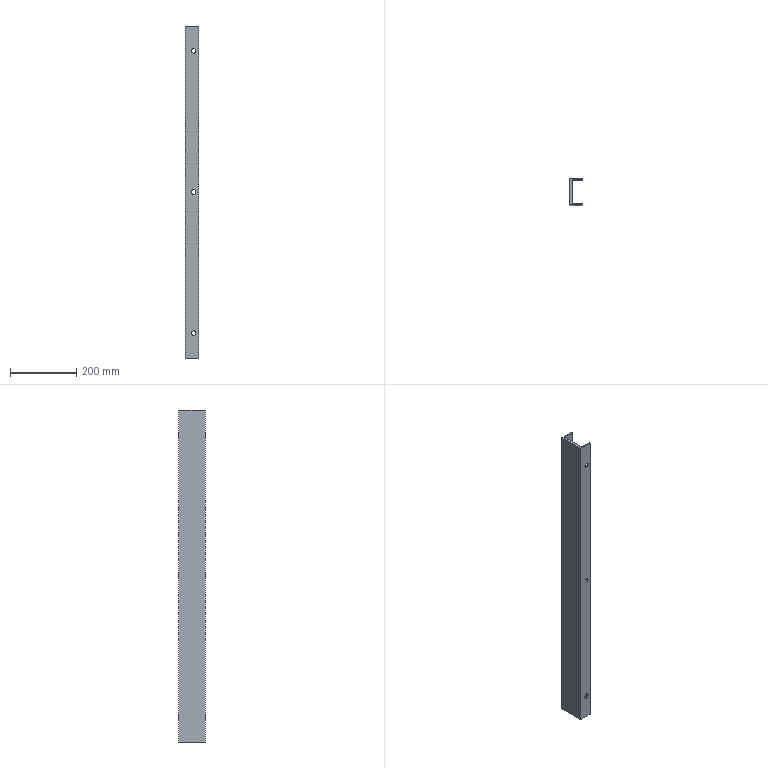Component | SolidWorks | BaseAssembly-1_ChannelSteelAssembly-1_8#ChannelSteel1-1 | 1 solid | 22 faces | box 40 x 80 x 1000 mm | volume 892305 mm3 | cylinder 12 | plane 10 | commonest cylinder face diameters 14 x12
build123d program:
from build123d import *

# Parameters (mm, degrees)
EXTRUDE1_DEPTH     = 1000
SKETCH2_R          = 7
CUT_EXTRUDE1_DEPTH = 1004.992
LPATTERN1_COUNT    = 3
LPATTERN1_PITCH    = 425


with BuildPart() as part:
    # Sketch1 → Extrude1 (new body)
    with BuildSketch(Plane.XY):
        Polygon((0, 0), (-40, 0), (-40, 80), (0, 80), (0, 76), (-32, 76), (-32, 4), (0, 4), align=None)
    extrude(amount=EXTRUDE1_DEPTH)

    # Sketch2 → Cut-Extrude1 (cut, through all)
    with BuildSketch(Plane(origin=(0, 80, 0), x_dir=(1, 0, 0), z_dir=(0, 1, 0))):
        with Locations(Location((-15, -925, 0), (0, 0, 270))):
            Circle(SKETCH2_R)
    cut_extrude1 = extrude(amount=-CUT_EXTRUDE1_DEPTH, mode=Mode.SUBTRACT)

    # LPattern1: Cut-Extrude1 ×3
    with Locations(*[(0, 0, -i * LPATTERN1_PITCH) for i in range(1, LPATTERN1_COUNT)]):
        add(cut_extrude1, mode=Mode.SUBTRACT)


solid = part.part

# Placed as in the assembly
solid = solid.moved(Location((-377.218, -82.9, -600), (0, 0, 0)))
STEP:
#1=COLOUR_RGB('',0.7922,0.8196,0.9333);
#2=FILL_AREA_STYLE_COLOUR('',#1);
#3=FILL_AREA_STYLE('',(#2));
#4=SURFACE_STYLE_FILL_AREA(#3);
#5=SURFACE_SIDE_STYLE('',(#4));
#6=SURFACE_STYLE_USAGE(.BOTH.,#5);
#7=PRESENTATION_STYLE_ASSIGNMENT((#6));
#8=CARTESIAN_POINT('',(-15.442,-3.264,-20.945));
#9=VERTEX_POINT('',#8);
#10=CARTESIAN_POINT('',(-15.442,-3.264,-20.394));
#11=VERTEX_POINT('',#10);
#12=CARTESIAN_POINT('',(-15.442,-3.264,-20.669));
#13=DIRECTION('',(0.,1.,0.));
#14=DIRECTION('',(0.,0.,1.));
#15=AXIS2_PLACEMENT_3D('',#12,#13,#14);
#16=CIRCLE('',#15,0.2756);
#17=EDGE_CURVE('',#9,#11,#16,.T.);
#18=ORIENTED_EDGE('',*,*,#17,.F.);
#19=CARTESIAN_POINT('',(-15.442,-3.106,-20.945));
#20=VERTEX_POINT('',#19);
#21=CARTESIAN_POINT('',(-15.442,-3.264,-20.945));
#22=DIRECTION('',(0.,1.,0.));
#23=VECTOR('',#22,39.37);
#24=LINE('',#21,#23);
#25=EDGE_CURVE('',#9,#20,#24,.T.);
#26=ORIENTED_EDGE('',*,*,#25,.T.);
#27=CARTESIAN_POINT('',(-15.442,-3.106,-20.394));
#28=VERTEX_POINT('',#27);
#29=CARTESIAN_POINT('',(-15.442,-3.106,-20.669));
#30=DIRECTION('',(0.,-1.,0.));
#31=DIRECTION('',(0.,0.,-1.));
#32=AXIS2_PLACEMENT_3D('',#29,#30,#31);
#33=CIRCLE('',#32,0.2756);
#34=EDGE_CURVE('',#28,#20,#33,.T.);
#35=ORIENTED_EDGE('',*,*,#34,.F.);
#36=CARTESIAN_POINT('',(-15.442,-3.264,-20.394));
#37=DIRECTION('',(0.,1.,0.));
#38=VECTOR('',#37,39.37);
#39=LINE('',#36,#38);
#40=EDGE_CURVE('',#11,#28,#39,.T.);
#41=ORIENTED_EDGE('',*,*,#40,.F.);
#42=EDGE_LOOP('',(#18,#26,#35,#41));
#43=FACE_OUTER_BOUND('',#42,.T.);
#44=CARTESIAN_POINT('',(-15.442,-3.264,-20.669));
#45=DIRECTION('',(0.,1.,0.));
#46=DIRECTION('',(0.,0.,1.));
#47=AXIS2_PLACEMENT_3D('',#44,#45,#46);
#48=CYLINDRICAL_SURFACE('',#47,0.2756);
#49=ADVANCED_FACE('',(#43),#48,.F.);
#50=CARTESIAN_POINT('',(-15.442,-3.264,-4.213));
#51=VERTEX_POINT('',#50);
#52=CARTESIAN_POINT('',(-15.442,-3.264,-3.661));
#53=VERTEX_POINT('',#52);
#54=CARTESIAN_POINT('',(-15.442,-3.264,-3.937));
#55=DIRECTION('',(0.,1.,0.));
#56=DIRECTION('',(0.,0.,1.));
#57=AXIS2_PLACEMENT_3D('',#54,#55,#56);
#58=CIRCLE('',#57,0.2756);
#59=EDGE_CURVE('',#51,#53,#58,.T.);
#60=ORIENTED_EDGE('',*,*,#59,.F.);
#61=CARTESIAN_POINT('',(-15.442,-3.106,-4.213));
#62=VERTEX_POINT('',#61);
#63=CARTESIAN_POINT('',(-15.442,-3.264,-4.213));
#64=DIRECTION('',(0.,1.,0.));
#65=VECTOR('',#64,39.37);
#66=LINE('',#63,#65);
#67=EDGE_CURVE('',#51,#62,#66,.T.);
#68=ORIENTED_EDGE('',*,*,#67,.T.);
#69=CARTESIAN_POINT('',(-15.442,-3.106,-3.661));
#70=VERTEX_POINT('',#69);
#71=CARTESIAN_POINT('',(-15.442,-3.106,-3.937));
#72=DIRECTION('',(0.,-1.,0.));
#73=DIRECTION('',(0.,0.,-1.));
#74=AXIS2_PLACEMENT_3D('',#71,#72,#73);
#75=CIRCLE('',#74,0.2756);
#76=EDGE_CURVE('',#70,#62,#75,.T.);
#77=ORIENTED_EDGE('',*,*,#76,.F.);
#78=CARTESIAN_POINT('',(-15.442,-3.264,-3.661));
#79=DIRECTION('',(0.,1.,0.));
#80=VECTOR('',#79,39.37);
#81=LINE('',#78,#80);
#82=EDGE_CURVE('',#53,#70,#81,.T.);
#83=ORIENTED_EDGE('',*,*,#82,.F.);
#84=EDGE_LOOP('',(#60,#68,#77,#83));
#85=FACE_OUTER_BOUND('',#84,.T.);
#86=CARTESIAN_POINT('',(-15.442,-3.264,-3.937));
#87=DIRECTION('',(0.,1.,0.));
#88=DIRECTION('',(0.,0.,1.));
#89=AXIS2_PLACEMENT_3D('',#86,#87,#88);
#90=CYLINDRICAL_SURFACE('',#89,0.2756);
#91=ADVANCED_FACE('',(#85),#90,.F.);
#92=CARTESIAN_POINT('',(-15.442,-0.2717,-20.945));
#93=VERTEX_POINT('',#92);
#94=CARTESIAN_POINT('',(-15.442,-0.2717,-20.394));
#95=VERTEX_POINT('',#94);
#96=CARTESIAN_POINT('',(-15.442,-0.2717,-20.669));
#97=DIRECTION('',(0.,1.,0.));
#98=DIRECTION('',(0.,0.,1.));
#99=AXIS2_PLACEMENT_3D('',#96,#97,#98);
#100=CIRCLE('',#99,0.2756);
#101=EDGE_CURVE('',#93,#95,#100,.T.);
#102=ORIENTED_EDGE('',*,*,#101,.F.);
#103=CARTESIAN_POINT('',(-15.442,-0.1142,-20.945));
#104=VERTEX_POINT('',#103);
#105=CARTESIAN_POINT('',(-15.442,-3.264,-20.945));
#106=DIRECTION('',(0.,1.,0.));
#107=VECTOR('',#106,39.37);
#108=LINE('',#105,#107);
#109=EDGE_CURVE('',#93,#104,#108,.T.);
#110=ORIENTED_EDGE('',*,*,#109,.T.);
#111=CARTESIAN_POINT('',(-15.442,-0.1142,-20.394));
#112=VERTEX_POINT('',#111);
#113=CARTESIAN_POINT('',(-15.442,-0.1142,-20.669));
#114=DIRECTION('',(0.,1.,0.));
#115=DIRECTION('',(0.,0.,1.));
#116=AXIS2_PLACEMENT_3D('',#113,#114,#115);
#117=CIRCLE('',#116,0.2756);
#118=EDGE_CURVE('',#104,#112,#117,.T.);
#119=ORIENTED_EDGE('',*,*,#118,.T.);
#120=CARTESIAN_POINT('',(-15.442,-3.264,-20.394));
#121=DIRECTION('',(0.,1.,0.));
#122=VECTOR('',#121,39.37);
#123=LINE('',#120,#122);
#124=EDGE_CURVE('',#95,#112,#123,.T.);
#125=ORIENTED_EDGE('',*,*,#124,.F.);
#126=EDGE_LOOP('',(#102,#110,#119,#125));
#127=FACE_OUTER_BOUND('',#126,.T.);
#128=CARTESIAN_POINT('',(-15.442,-3.264,-20.669));
#129=DIRECTION('',(0.,1.,0.));
#130=DIRECTION('',(0.,0.,1.));
#131=AXIS2_PLACEMENT_3D('',#128,#129,#130);
#132=CYLINDRICAL_SURFACE('',#131,0.2756);
#133=ADVANCED_FACE('',(#127),#132,.F.);
#134=CARTESIAN_POINT('',(-15.442,-0.2717,-4.213));
#135=VERTEX_POINT('',#134);
#136=CARTESIAN_POINT('',(-15.442,-0.2717,-3.661));
#137=VERTEX_POINT('',#136);
#138=CARTESIAN_POINT('',(-15.442,-0.2717,-3.937));
#139=DIRECTION('',(0.,1.,0.));
#140=DIRECTION('',(0.,0.,1.));
#141=AXIS2_PLACEMENT_3D('',#138,#139,#140);
#142=CIRCLE('',#141,0.2756);
#143=EDGE_CURVE('',#135,#137,#142,.T.);
#144=ORIENTED_EDGE('',*,*,#143,.F.);
#145=CARTESIAN_POINT('',(-15.442,-0.1142,-4.213));
#146=VERTEX_POINT('',#145);
#147=CARTESIAN_POINT('',(-15.442,-3.264,-4.213));
#148=DIRECTION('',(0.,1.,0.));
#149=VECTOR('',#148,39.37);
#150=LINE('',#147,#149);
#151=EDGE_CURVE('',#135,#146,#150,.T.);
#152=ORIENTED_EDGE('',*,*,#151,.T.);
#153=CARTESIAN_POINT('',(-15.442,-0.1142,-3.661));
#154=VERTEX_POINT('',#153);
#155=CARTESIAN_POINT('',(-15.442,-0.1142,-3.937));
#156=DIRECTION('',(0.,1.,0.));
#157=DIRECTION('',(0.,0.,1.));
#158=AXIS2_PLACEMENT_3D('',#155,#156,#157);
#159=CIRCLE('',#158,0.2756);
#160=EDGE_CURVE('',#146,#154,#159,.T.);
#161=ORIENTED_EDGE('',*,*,#160,.T.);
#162=CARTESIAN_POINT('',(-15.442,-3.264,-3.661));
#163=DIRECTION('',(0.,1.,0.));
#164=VECTOR('',#163,39.37);
#165=LINE('',#162,#164);
#166=EDGE_CURVE('',#137,#154,#165,.T.);
#167=ORIENTED_EDGE('',*,*,#166,.F.);
#168=EDGE_LOOP('',(#144,#152,#161,#167));
#169=FACE_OUTER_BOUND('',#168,.T.);
#170=CARTESIAN_POINT('',(-15.442,-3.264,-3.937));
#171=DIRECTION('',(0.,1.,0.));
#172=DIRECTION('',(0.,0.,1.));
#173=AXIS2_PLACEMENT_3D('',#170,#171,#172);
#174=CYLINDRICAL_SURFACE('',#173,0.2756);
#175=ADVANCED_FACE('',(#169),#174,.F.);
#176=CARTESIAN_POINT('',(-15.442,-0.2717,12.52));
#177=VERTEX_POINT('',#176);
#178=CARTESIAN_POINT('',(-15.442,-0.2717,13.071));
#179=VERTEX_POINT('',#178);
#180=CARTESIAN_POINT('',(-15.442,-0.2717,12.795));
#181=DIRECTION('',(0.,1.,0.));
#182=DIRECTION('',(0.,0.,1.));
#183=AXIS2_PLACEMENT_3D('',#180,#181,#182);
#184=CIRCLE('',#183,0.2756);
#185=EDGE_CURVE('',#177,#179,#184,.T.);
#186=ORIENTED_EDGE('',*,*,#185,.F.);
#187=CARTESIAN_POINT('',(-15.442,-0.1142,12.52));
#188=VERTEX_POINT('',#187);
#189=CARTESIAN_POINT('',(-15.442,-3.264,12.52));
#190=DIRECTION('',(0.,1.,0.));
#191=VECTOR('',#190,39.37);
#192=LINE('',#189,#191);
#193=EDGE_CURVE('',#177,#188,#192,.T.);
#194=ORIENTED_EDGE('',*,*,#193,.T.);
#195=CARTESIAN_POINT('',(-15.442,-0.1142,13.071));
#196=VERTEX_POINT('',#195);
#197=CARTESIAN_POINT('',(-15.442,-0.1142,12.795));
#198=DIRECTION('',(0.,1.,0.));
#199=DIRECTION('',(0.,0.,1.));
#200=AXIS2_PLACEMENT_3D('',#197,#198,#199);
#201=CIRCLE('',#200,0.2756);
#202=EDGE_CURVE('',#188,#196,#201,.T.);
#203=ORIENTED_EDGE('',*,*,#202,.T.);
#204=CARTESIAN_POINT('',(-15.442,-3.264,13.071));
#205=DIRECTION('',(0.,1.,0.));
#206=VECTOR('',#205,39.37);
#207=LINE('',#204,#206);
#208=EDGE_CURVE('',#179,#196,#207,.T.);
#209=ORIENTED_EDGE('',*,*,#208,.F.);
#210=EDGE_LOOP('',(#186,#194,#203,#209));
#211=FACE_OUTER_BOUND('',#210,.T.);
#212=CARTESIAN_POINT('',(-15.442,-3.264,12.795));
#213=DIRECTION('',(0.,1.,0.));
#214=DIRECTION('',(0.,0.,1.));
#215=AXIS2_PLACEMENT_3D('',#212,#213,#214);
#216=CYLINDRICAL_SURFACE('',#215,0.2756);
#217=ADVANCED_FACE('',(#211),#216,.F.);
#218=CARTESIAN_POINT('',(-15.442,-3.264,12.52));
#219=VERTEX_POINT('',#218);
#220=CARTESIAN_POINT('',(-15.442,-3.264,13.071));
#221=VERTEX_POINT('',#220);
#222=CARTESIAN_POINT('',(-15.442,-3.264,12.795));
#223=DIRECTION('',(0.,1.,0.));
#224=DIRECTION('',(0.,0.,1.));
#225=AXIS2_PLACEMENT_3D('',#222,#223,#224);
#226=CIRCLE('',#225,0.2756);
#227=EDGE_CURVE('',#219,#221,#226,.T.);
#228=ORIENTED_EDGE('',*,*,#227,.F.);
#229=CARTESIAN_POINT('',(-15.442,-3.106,12.52));
#230=VERTEX_POINT('',#229);
#231=CARTESIAN_POINT('',(-15.442,-3.264,12.52));
#232=DIRECTION('',(0.,1.,0.));
#233=VECTOR('',#232,39.37);
#234=LINE('',#231,#233);
#235=EDGE_CURVE('',#219,#230,#234,.T.);
#236=ORIENTED_EDGE('',*,*,#235,.T.);
#237=CARTESIAN_POINT('',(-15.442,-3.106,13.071));
#238=VERTEX_POINT('',#237);
#239=CARTESIAN_POINT('',(-15.442,-3.106,12.795));
#240=DIRECTION('',(0.,-1.,0.));
#241=DIRECTION('',(0.,0.,-1.));
#242=AXIS2_PLACEMENT_3D('',#239,#240,#241);
#243=CIRCLE('',#242,0.2756);
#244=EDGE_CURVE('',#238,#230,#243,.T.);
#245=ORIENTED_EDGE('',*,*,#244,.F.);
#246=CARTESIAN_POINT('',(-15.442,-3.264,13.071));
#247=DIRECTION('',(0.,1.,0.));
#248=VECTOR('',#247,39.37);
#249=LINE('',#246,#248);
#250=EDGE_CURVE('',#221,#238,#249,.T.);
#251=ORIENTED_EDGE('',*,*,#250,.F.);
#252=EDGE_LOOP('',(#228,#236,#245,#251));
#253=FACE_OUTER_BOUND('',#252,.T.);
#254=CARTESIAN_POINT('',(-15.442,-3.264,12.795));
#255=DIRECTION('',(0.,1.,0.));
#256=DIRECTION('',(0.,0.,1.));
#257=AXIS2_PLACEMENT_3D('',#254,#255,#256);
#258=CYLINDRICAL_SURFACE('',#257,0.2756);
#259=ADVANCED_FACE('',(#253),#258,.F.);
#260=CARTESIAN_POINT('',(-14.851,-3.264,-23.622));
#261=VERTEX_POINT('',#260);
#262=CARTESIAN_POINT('',(-14.851,-3.106,-23.622));
#263=VERTEX_POINT('',#262);
#264=CARTESIAN_POINT('',(-14.851,-3.106,-23.622));
#265=DIRECTION('',(0.,1.,0.));
#266=VECTOR('',#265,39.37);
#267=LINE('',#264,#266);
#268=EDGE_CURVE('',#261,#263,#267,.T.);
#269=ORIENTED_EDGE('',*,*,#268,.T.);
#270=CARTESIAN_POINT('',(-14.851,-3.106,15.748));
#271=VERTEX_POINT('',#270);
#272=CARTESIAN_POINT('',(-14.851,-3.106,15.748));
#273=DIRECTION('',(0.,0.,-1.));
#274=VECTOR('',#273,39.37);
#275=LINE('',#272,#274);
#276=EDGE_CURVE('',#271,#263,#275,.T.);
#277=ORIENTED_EDGE('',*,*,#276,.F.);
#278=CARTESIAN_POINT('',(-14.851,-3.264,15.748));
#279=VERTEX_POINT('',#278);
#280=CARTESIAN_POINT('',(-14.851,-3.106,15.748));
#281=DIRECTION('',(0.,1.,0.));
#282=VECTOR('',#281,39.37);
#283=LINE('',#280,#282);
#284=EDGE_CURVE('',#279,#271,#283,.T.);
#285=ORIENTED_EDGE('',*,*,#284,.F.);
#286=CARTESIAN_POINT('',(-14.851,-3.264,15.748));
#287=DIRECTION('',(0.,0.,-1.));
#288=VECTOR('',#287,39.37);
#289=LINE('',#286,#288);
#290=EDGE_CURVE('',#279,#261,#289,.T.);
#291=ORIENTED_EDGE('',*,*,#290,.T.);
#292=EDGE_LOOP('',(#269,#277,#285,#291));
#293=FACE_OUTER_BOUND('',#292,.T.);
#294=CARTESIAN_POINT('',(-14.851,-3.106,15.748));
#295=DIRECTION('',(-1.,0.,0.));
#296=DIRECTION('',(-0.,-1.,0.));
#297=AXIS2_PLACEMENT_3D('',#294,#295,#296);
#298=PLANE('',#297);
#299=ADVANCED_FACE('',(#293),#298,.F.);
#300=ORIENTED_EDGE('',*,*,#76,.T.);
#301=CARTESIAN_POINT('',(-15.442,-3.106,-3.937));
#302=DIRECTION('',(0.,-1.,0.));
#303=DIRECTION('',(0.,0.,-1.));
#304=AXIS2_PLACEMENT_3D('',#301,#302,#303);
#305=CIRCLE('',#304,0.2756);
#306=EDGE_CURVE('',#62,#70,#305,.T.);
#307=ORIENTED_EDGE('',*,*,#306,.T.);
#308=EDGE_LOOP('',(#300,#307));
#309=FACE_BOUND('',#308,.T.);
#310=ORIENTED_EDGE('',*,*,#244,.T.);
#311=CARTESIAN_POINT('',(-15.442,-3.106,12.795));
#312=DIRECTION('',(0.,-1.,0.));
#313=DIRECTION('',(0.,0.,-1.));
#314=AXIS2_PLACEMENT_3D('',#311,#312,#313);
#315=CIRCLE('',#314,0.2756);
#316=EDGE_CURVE('',#230,#238,#315,.T.);
#317=ORIENTED_EDGE('',*,*,#316,.T.);
#318=EDGE_LOOP('',(#310,#317));
#319=FACE_BOUND('',#318,.T.);
#320=CARTESIAN_POINT('',(-16.111,-3.106,-23.622));
#321=VERTEX_POINT('',#320);
#322=CARTESIAN_POINT('',(-16.111,-3.106,-23.622));
#323=DIRECTION('',(-1.,0.,0.));
#324=VECTOR('',#323,39.37);
#325=LINE('',#322,#324);
#326=EDGE_CURVE('',#263,#321,#325,.T.);
#327=ORIENTED_EDGE('',*,*,#326,.T.);
#328=CARTESIAN_POINT('',(-16.111,-3.106,15.748));
#329=VERTEX_POINT('',#328);
#330=CARTESIAN_POINT('',(-16.111,-3.106,15.748));
#331=DIRECTION('',(0.,0.,-1.));
#332=VECTOR('',#331,39.37);
#333=LINE('',#330,#332);
#334=EDGE_CURVE('',#329,#321,#333,.T.);
#335=ORIENTED_EDGE('',*,*,#334,.F.);
#336=CARTESIAN_POINT('',(-16.111,-3.106,15.748));
#337=DIRECTION('',(-1.,0.,0.));
#338=VECTOR('',#337,39.37);
#339=LINE('',#336,#338);
#340=EDGE_CURVE('',#271,#329,#339,.T.);
#341=ORIENTED_EDGE('',*,*,#340,.F.);
#342=ORIENTED_EDGE('',*,*,#276,.T.);
#343=EDGE_LOOP('',(#327,#335,#341,#342));
#344=FACE_OUTER_BOUND('',#343,.T.);
#345=ORIENTED_EDGE('',*,*,#34,.T.);
#346=CARTESIAN_POINT('',(-15.442,-3.106,-20.669));
#347=DIRECTION('',(0.,-1.,0.));
#348=DIRECTION('',(0.,0.,-1.));
#349=AXIS2_PLACEMENT_3D('',#346,#347,#348);
#350=CIRCLE('',#349,0.2756);
#351=EDGE_CURVE('',#20,#28,#350,.T.);
#352=ORIENTED_EDGE('',*,*,#351,.T.);
#353=EDGE_LOOP('',(#345,#352));
#354=FACE_BOUND('',#353,.T.);
#355=CARTESIAN_POINT('',(-16.111,-3.106,15.748));
#356=DIRECTION('',(0.,-1.,0.));
#357=DIRECTION('',(0.,0.,-1.));
#358=AXIS2_PLACEMENT_3D('',#355,#356,#357);
#359=PLANE('',#358);
#360=ADVANCED_FACE('',(#309,#319,#344,#354),#359,.F.);
#361=CARTESIAN_POINT('',(-16.111,-0.2717,-23.622));
#362=VERTEX_POINT('',#361);
#363=CARTESIAN_POINT('',(-16.111,-0.2717,-23.622));
#364=DIRECTION('',(-0.,1.,0.));
#365=VECTOR('',#364,39.37);
#366=LINE('',#363,#365);
#367=EDGE_CURVE('',#321,#362,#366,.T.);
#368=ORIENTED_EDGE('',*,*,#367,.T.);
#369=CARTESIAN_POINT('',(-16.111,-0.2717,15.748));
#370=VERTEX_POINT('',#369);
#371=CARTESIAN_POINT('',(-16.111,-0.2717,15.748));
#372=DIRECTION('',(0.,0.,-1.));
#373=VECTOR('',#372,39.37);
#374=LINE('',#371,#373);
#375=EDGE_CURVE('',#370,#362,#374,.T.);
#376=ORIENTED_EDGE('',*,*,#375,.F.);
#377=CARTESIAN_POINT('',(-16.111,-0.2717,15.748));
#378=DIRECTION('',(-0.,1.,0.));
#379=VECTOR('',#378,39.37);
#380=LINE('',#377,#379);
#381=EDGE_CURVE('',#329,#370,#380,.T.);
#382=ORIENTED_EDGE('',*,*,#381,.F.);
#383=ORIENTED_EDGE('',*,*,#334,.T.);
#384=EDGE_LOOP('',(#368,#376,#382,#383));
#385=FACE_OUTER_BOUND('',#384,.T.);
#386=CARTESIAN_POINT('',(-16.111,-0.2717,15.748));
#387=DIRECTION('',(-1.,-0.,0.));
#388=DIRECTION('',(0.,-1.,0.));
#389=AXIS2_PLACEMENT_3D('',#386,#387,#388);
#390=PLANE('',#389);
#391=ADVANCED_FACE('',(#385),#390,.F.);
#392=CARTESIAN_POINT('',(-15.442,-0.2717,-3.937));
#393=DIRECTION('',(0.,1.,0.));
#394=DIRECTION('',(0.,0.,1.));
#395=AXIS2_PLACEMENT_3D('',#392,#393,#394);
#396=CIRCLE('',#395,0.2756);
#397=EDGE_CURVE('',#137,#135,#396,.T.);
#398=ORIENTED_EDGE('',*,*,#397,.T.);
#399=ORIENTED_EDGE('',*,*,#143,.T.);
#400=EDGE_LOOP('',(#398,#399));
#401=FACE_BOUND('',#400,.T.);
#402=CARTESIAN_POINT('',(-15.442,-0.2717,12.795));
#403=DIRECTION('',(0.,1.,0.));
#404=DIRECTION('',(0.,0.,1.));
#405=AXIS2_PLACEMENT_3D('',#402,#403,#404);
#406=CIRCLE('',#405,0.2756);
#407=EDGE_CURVE('',#179,#177,#406,.T.);
#408=ORIENTED_EDGE('',*,*,#407,.T.);
#409=ORIENTED_EDGE('',*,*,#185,.T.);
#410=EDGE_LOOP('',(#408,#409));
#411=FACE_BOUND('',#410,.T.);
#412=CARTESIAN_POINT('',(-14.851,-0.2717,-23.622));
#413=VERTEX_POINT('',#412);
#414=CARTESIAN_POINT('',(-14.851,-0.2717,-23.622));
#415=DIRECTION('',(1.,0.,0.));
#416=VECTOR('',#415,39.37);
#417=LINE('',#414,#416);
#418=EDGE_CURVE('',#362,#413,#417,.T.);
#419=ORIENTED_EDGE('',*,*,#418,.T.);
#420=CARTESIAN_POINT('',(-14.851,-0.2717,15.748));
#421=VERTEX_POINT('',#420);
#422=CARTESIAN_POINT('',(-14.851,-0.2717,15.748));
#423=DIRECTION('',(0.,0.,-1.));
#424=VECTOR('',#423,39.37);
#425=LINE('',#422,#424);
#426=EDGE_CURVE('',#421,#413,#425,.T.);
#427=ORIENTED_EDGE('',*,*,#426,.F.);
#428=CARTESIAN_POINT('',(-14.851,-0.2717,15.748));
#429=DIRECTION('',(1.,0.,0.));
#430=VECTOR('',#429,39.37);
#431=LINE('',#428,#430);
#432=EDGE_CURVE('',#370,#421,#431,.T.);
#433=ORIENTED_EDGE('',*,*,#432,.F.);
#434=ORIENTED_EDGE('',*,*,#375,.T.);
#435=EDGE_LOOP('',(#419,#427,#433,#434));
#436=FACE_OUTER_BOUND('',#435,.T.);
#437=CARTESIAN_POINT('',(-15.442,-0.2717,-20.669));
#438=DIRECTION('',(0.,1.,0.));
#439=DIRECTION('',(0.,0.,1.));
#440=AXIS2_PLACEMENT_3D('',#437,#438,#439);
#441=CIRCLE('',#440,0.2756);
#442=EDGE_CURVE('',#95,#93,#441,.T.);
#443=ORIENTED_EDGE('',*,*,#442,.T.);
#444=ORIENTED_EDGE('',*,*,#101,.T.);
#445=EDGE_LOOP('',(#443,#444));
#446=FACE_BOUND('',#445,.T.);
#447=CARTESIAN_POINT('',(-14.851,-0.2717,15.748));
#448=DIRECTION('',(0.,1.,0.));
#449=DIRECTION('',(0.,0.,1.));
#450=AXIS2_PLACEMENT_3D('',#447,#448,#449);
#451=PLANE('',#450);
#452=ADVANCED_FACE('',(#401,#411,#436,#446),#451,.F.);
#453=CARTESIAN_POINT('',(-14.851,-0.1142,-23.622));
#454=VERTEX_POINT('',#453);
#455=CARTESIAN_POINT('',(-14.851,-0.1142,-23.622));
#456=DIRECTION('',(0.,1.,0.));
#457=VECTOR('',#456,39.37);
#458=LINE('',#455,#457);
#459=EDGE_CURVE('',#413,#454,#458,.T.);
#460=ORIENTED_EDGE('',*,*,#459,.T.);
#461=CARTESIAN_POINT('',(-14.851,-0.1142,15.748));
#462=VERTEX_POINT('',#461);
#463=CARTESIAN_POINT('',(-14.851,-0.1142,15.748));
#464=DIRECTION('',(0.,0.,-1.));
#465=VECTOR('',#464,39.37);
#466=LINE('',#463,#465);
#467=EDGE_CURVE('',#462,#454,#466,.T.);
#468=ORIENTED_EDGE('',*,*,#467,.F.);
#469=CARTESIAN_POINT('',(-14.851,-0.1142,15.748));
#470=DIRECTION('',(0.,1.,0.));
#471=VECTOR('',#470,39.37);
#472=LINE('',#469,#471);
#473=EDGE_CURVE('',#421,#462,#472,.T.);
#474=ORIENTED_EDGE('',*,*,#473,.F.);
#475=ORIENTED_EDGE('',*,*,#426,.T.);
#476=EDGE_LOOP('',(#460,#468,#474,#475));
#477=FACE_OUTER_BOUND('',#476,.T.);
#478=CARTESIAN_POINT('',(-14.851,-0.1142,15.748));
#479=DIRECTION('',(-1.,0.,0.));
#480=DIRECTION('',(0.,0.,1.));
#481=AXIS2_PLACEMENT_3D('',#478,#479,#480);
#482=PLANE('',#481);
#483=ADVANCED_FACE('',(#477),#482,.F.);
#484=CARTESIAN_POINT('',(-15.442,-0.1142,-3.937));
#485=DIRECTION('',(0.,1.,0.));
#486=DIRECTION('',(0.,0.,1.));
#487=AXIS2_PLACEMENT_3D('',#484,#485,#486);
#488=CIRCLE('',#487,0.2756);
#489=EDGE_CURVE('',#154,#146,#488,.T.);
#490=ORIENTED_EDGE('',*,*,#489,.F.);
#491=ORIENTED_EDGE('',*,*,#160,.F.);
#492=EDGE_LOOP('',(#490,#491));
#493=FACE_BOUND('',#492,.T.);
#494=CARTESIAN_POINT('',(-15.442,-0.1142,12.795));
#495=DIRECTION('',(0.,1.,0.));
#496=DIRECTION('',(0.,0.,1.));
#497=AXIS2_PLACEMENT_3D('',#494,#495,#496);
#498=CIRCLE('',#497,0.2756);
#499=EDGE_CURVE('',#196,#188,#498,.T.);
#500=ORIENTED_EDGE('',*,*,#499,.F.);
#501=ORIENTED_EDGE('',*,*,#202,.F.);
#502=EDGE_LOOP('',(#500,#501));
#503=FACE_BOUND('',#502,.T.);
#504=CARTESIAN_POINT('',(-16.426,-0.1142,-23.622));
#505=VERTEX_POINT('',#504);
#506=CARTESIAN_POINT('',(-16.426,-0.1142,-23.622));
#507=DIRECTION('',(-1.,0.,0.));
#508=VECTOR('',#507,39.37);
#509=LINE('',#506,#508);
#510=EDGE_CURVE('',#454,#505,#509,.T.);
#511=ORIENTED_EDGE('',*,*,#510,.T.);
#512=CARTESIAN_POINT('',(-16.426,-0.1142,15.748));
#513=VERTEX_POINT('',#512);
#514=CARTESIAN_POINT('',(-16.426,-0.1142,15.748));
#515=DIRECTION('',(0.,0.,-1.));
#516=VECTOR('',#515,39.37);
#517=LINE('',#514,#516);
#518=EDGE_CURVE('',#513,#505,#517,.T.);
#519=ORIENTED_EDGE('',*,*,#518,.F.);
#520=CARTESIAN_POINT('',(-16.426,-0.1142,15.748));
#521=DIRECTION('',(-1.,0.,0.));
#522=VECTOR('',#521,39.37);
#523=LINE('',#520,#522);
#524=EDGE_CURVE('',#462,#513,#523,.T.);
#525=ORIENTED_EDGE('',*,*,#524,.F.);
#526=ORIENTED_EDGE('',*,*,#467,.T.);
#527=EDGE_LOOP('',(#511,#519,#525,#526));
#528=FACE_OUTER_BOUND('',#527,.T.);
#529=CARTESIAN_POINT('',(-15.442,-0.1142,-20.669));
#530=DIRECTION('',(0.,1.,0.));
#531=DIRECTION('',(0.,0.,1.));
#532=AXIS2_PLACEMENT_3D('',#529,#530,#531);
#533=CIRCLE('',#532,0.2756);
#534=EDGE_CURVE('',#112,#104,#533,.T.);
#535=ORIENTED_EDGE('',*,*,#534,.F.);
#536=ORIENTED_EDGE('',*,*,#118,.F.);
#537=EDGE_LOOP('',(#535,#536));
#538=FACE_BOUND('',#537,.T.);
#539=CARTESIAN_POINT('',(-16.426,-0.1142,15.748));
#540=DIRECTION('',(0.,-1.,0.));
#541=DIRECTION('',(0.,0.,-1.));
#542=AXIS2_PLACEMENT_3D('',#539,#540,#541);
#543=PLANE('',#542);
#544=ADVANCED_FACE('',(#493,#503,#528,#538),#543,.F.);
#545=CARTESIAN_POINT('',(-16.426,-3.264,-23.622));
#546=VERTEX_POINT('',#545);
#547=CARTESIAN_POINT('',(-16.426,-3.264,-23.622));
#548=DIRECTION('',(0.,-1.,0.));
#549=VECTOR('',#548,39.37);
#550=LINE('',#547,#549);
#551=EDGE_CURVE('',#505,#546,#550,.T.);
#552=ORIENTED_EDGE('',*,*,#551,.T.);
#553=CARTESIAN_POINT('',(-16.426,-3.264,15.748));
#554=VERTEX_POINT('',#553);
#555=CARTESIAN_POINT('',(-16.426,-3.264,15.748));
#556=DIRECTION('',(0.,0.,-1.));
#557=VECTOR('',#556,39.37);
#558=LINE('',#555,#557);
#559=EDGE_CURVE('',#554,#546,#558,.T.);
#560=ORIENTED_EDGE('',*,*,#559,.F.);
#561=CARTESIAN_POINT('',(-16.426,-3.264,15.748));
#562=DIRECTION('',(0.,-1.,0.));
#563=VECTOR('',#562,39.37);
#564=LINE('',#561,#563);
#565=EDGE_CURVE('',#513,#554,#564,.T.);
#566=ORIENTED_EDGE('',*,*,#565,.F.);
#567=ORIENTED_EDGE('',*,*,#518,.T.);
#568=EDGE_LOOP('',(#552,#560,#566,#567));
#569=FACE_OUTER_BOUND('',#568,.T.);
#570=CARTESIAN_POINT('',(-16.426,-3.264,15.748));
#571=DIRECTION('',(1.,0.,0.));
#572=DIRECTION('',(0.,0.,-1.));
#573=AXIS2_PLACEMENT_3D('',#570,#571,#572);
#574=PLANE('',#573);
#575=ADVANCED_FACE('',(#569),#574,.F.);
#576=CARTESIAN_POINT('',(-15.442,-3.264,-3.937));
#577=DIRECTION('',(0.,1.,0.));
#578=DIRECTION('',(0.,0.,1.));
#579=AXIS2_PLACEMENT_3D('',#576,#577,#578);
#580=CIRCLE('',#579,0.2756);
#581=EDGE_CURVE('',#53,#51,#580,.T.);
#582=ORIENTED_EDGE('',*,*,#581,.T.);
#583=ORIENTED_EDGE('',*,*,#59,.T.);
#584=EDGE_LOOP('',(#582,#583));
#585=FACE_BOUND('',#584,.T.);
#586=CARTESIAN_POINT('',(-15.442,-3.264,12.795));
#587=DIRECTION('',(0.,1.,0.));
#588=DIRECTION('',(0.,0.,1.));
#589=AXIS2_PLACEMENT_3D('',#586,#587,#588);
#590=CIRCLE('',#589,0.2756);
#591=EDGE_CURVE('',#221,#219,#590,.T.);
#592=ORIENTED_EDGE('',*,*,#591,.T.);
#593=ORIENTED_EDGE('',*,*,#227,.T.);
#594=EDGE_LOOP('',(#592,#593));
#595=FACE_BOUND('',#594,.T.);
#596=CARTESIAN_POINT('',(-14.851,-3.264,-23.622));
#597=DIRECTION('',(1.,0.,0.));
#598=VECTOR('',#597,39.37);
#599=LINE('',#596,#598);
#600=EDGE_CURVE('',#546,#261,#599,.T.);
#601=ORIENTED_EDGE('',*,*,#600,.T.);
#602=ORIENTED_EDGE('',*,*,#290,.F.);
#603=CARTESIAN_POINT('',(-14.851,-3.264,15.748));
#604=DIRECTION('',(1.,0.,0.));
#605=VECTOR('',#604,39.37);
#606=LINE('',#603,#605);
#607=EDGE_CURVE('',#554,#279,#606,.T.);
#608=ORIENTED_EDGE('',*,*,#607,.F.);
#609=ORIENTED_EDGE('',*,*,#559,.T.);
#610=EDGE_LOOP('',(#601,#602,#608,#609));
#611=FACE_OUTER_BOUND('',#610,.T.);
#612=CARTESIAN_POINT('',(-15.442,-3.264,-20.669));
#613=DIRECTION('',(0.,1.,0.));
#614=DIRECTION('',(0.,0.,1.));
#615=AXIS2_PLACEMENT_3D('',#612,#613,#614);
#616=CIRCLE('',#615,0.2756);
#617=EDGE_CURVE('',#11,#9,#616,.T.);
#618=ORIENTED_EDGE('',*,*,#617,.T.);
#619=ORIENTED_EDGE('',*,*,#17,.T.);
#620=EDGE_LOOP('',(#618,#619));
#621=FACE_BOUND('',#620,.T.);
#622=CARTESIAN_POINT('',(-14.851,-3.264,15.748));
#623=DIRECTION('',(-0.,1.,0.));
#624=DIRECTION('',(-1.,-0.,0.));
#625=AXIS2_PLACEMENT_3D('',#622,#623,#624);
#626=PLANE('',#625);
#627=ADVANCED_FACE('',(#585,#595,#611,#621),#626,.F.);
#628=ORIENTED_EDGE('',*,*,#284,.T.);
#629=ORIENTED_EDGE('',*,*,#340,.T.);
#630=ORIENTED_EDGE('',*,*,#381,.T.);
#631=ORIENTED_EDGE('',*,*,#432,.T.);
#632=ORIENTED_EDGE('',*,*,#473,.T.);
#633=ORIENTED_EDGE('',*,*,#524,.T.);
#634=ORIENTED_EDGE('',*,*,#565,.T.);
#635=ORIENTED_EDGE('',*,*,#607,.T.);
#636=EDGE_LOOP('',(#628,#629,#630,#631,#632,#633,#634,#635));
#637=FACE_OUTER_BOUND('',#636,.T.);
#638=CARTESIAN_POINT('',(-14.851,-0.1142,15.748));
#639=DIRECTION('',(0.,0.,1.));
#640=DIRECTION('',(1.,0.,0.));
#641=AXIS2_PLACEMENT_3D('',#638,#639,#640);
#642=PLANE('',#641);
#643=ADVANCED_FACE('',(#637),#642,.T.);
#644=ORIENTED_EDGE('',*,*,#268,.F.);
#645=ORIENTED_EDGE('',*,*,#600,.F.);
#646=ORIENTED_EDGE('',*,*,#551,.F.);
#647=ORIENTED_EDGE('',*,*,#510,.F.);
#648=ORIENTED_EDGE('',*,*,#459,.F.);
#649=ORIENTED_EDGE('',*,*,#418,.F.);
#650=ORIENTED_EDGE('',*,*,#367,.F.);
#651=ORIENTED_EDGE('',*,*,#326,.F.);
#652=EDGE_LOOP('',(#644,#645,#646,#647,#648,#649,#650,#651));
#653=FACE_OUTER_BOUND('',#652,.T.);
#654=CARTESIAN_POINT('',(-14.851,-0.1142,-23.622));
#655=DIRECTION('',(0.,0.,1.));
#656=DIRECTION('',(1.,0.,0.));
#657=AXIS2_PLACEMENT_3D('',#654,#655,#656);
#658=PLANE('',#657);
#659=ADVANCED_FACE('',(#653),#658,.F.);
#660=ORIENTED_EDGE('',*,*,#235,.F.);
#661=ORIENTED_EDGE('',*,*,#591,.F.);
#662=ORIENTED_EDGE('',*,*,#250,.T.);
#663=ORIENTED_EDGE('',*,*,#316,.F.);
#664=EDGE_LOOP('',(#660,#661,#662,#663));
#665=FACE_OUTER_BOUND('',#664,.T.);
#666=CARTESIAN_POINT('',(-15.442,-3.264,12.795));
#667=DIRECTION('',(0.,1.,0.));
#668=DIRECTION('',(0.,0.,1.));
#669=AXIS2_PLACEMENT_3D('',#666,#667,#668);
#670=CYLINDRICAL_SURFACE('',#669,0.2756);
#671=ADVANCED_FACE('',(#665),#670,.F.);
#672=ORIENTED_EDGE('',*,*,#193,.F.);
#673=ORIENTED_EDGE('',*,*,#407,.F.);
#674=ORIENTED_EDGE('',*,*,#208,.T.);
#675=ORIENTED_EDGE('',*,*,#499,.T.);
#676=EDGE_LOOP('',(#672,#673,#674,#675));
#677=FACE_OUTER_BOUND('',#676,.T.);
#678=CARTESIAN_POINT('',(-15.442,-3.264,12.795));
#679=DIRECTION('',(0.,1.,0.));
#680=DIRECTION('',(0.,0.,1.));
#681=AXIS2_PLACEMENT_3D('',#678,#679,#680);
#682=CYLINDRICAL_SURFACE('',#681,0.2756);
#683=ADVANCED_FACE('',(#677),#682,.F.);
#684=ORIENTED_EDGE('',*,*,#151,.F.);
#685=ORIENTED_EDGE('',*,*,#397,.F.);
#686=ORIENTED_EDGE('',*,*,#166,.T.);
#687=ORIENTED_EDGE('',*,*,#489,.T.);
#688=EDGE_LOOP('',(#684,#685,#686,#687));
#689=FACE_OUTER_BOUND('',#688,.T.);
#690=CARTESIAN_POINT('',(-15.442,-3.264,-3.937));
#691=DIRECTION('',(0.,1.,0.));
#692=DIRECTION('',(0.,0.,1.));
#693=AXIS2_PLACEMENT_3D('',#690,#691,#692);
#694=CYLINDRICAL_SURFACE('',#693,0.2756);
#695=ADVANCED_FACE('',(#689),#694,.F.);
#696=ORIENTED_EDGE('',*,*,#109,.F.);
#697=ORIENTED_EDGE('',*,*,#442,.F.);
#698=ORIENTED_EDGE('',*,*,#124,.T.);
#699=ORIENTED_EDGE('',*,*,#534,.T.);
#700=EDGE_LOOP('',(#696,#697,#698,#699));
#701=FACE_OUTER_BOUND('',#700,.T.);
#702=CARTESIAN_POINT('',(-15.442,-3.264,-20.669));
#703=DIRECTION('',(0.,1.,0.));
#704=DIRECTION('',(0.,0.,1.));
#705=AXIS2_PLACEMENT_3D('',#702,#703,#704);
#706=CYLINDRICAL_SURFACE('',#705,0.2756);
#707=ADVANCED_FACE('',(#701),#706,.F.);
#708=ORIENTED_EDGE('',*,*,#67,.F.);
#709=ORIENTED_EDGE('',*,*,#581,.F.);
#710=ORIENTED_EDGE('',*,*,#82,.T.);
#711=ORIENTED_EDGE('',*,*,#306,.F.);
#712=EDGE_LOOP('',(#708,#709,#710,#711));
#713=FACE_OUTER_BOUND('',#712,.T.);
#714=CARTESIAN_POINT('',(-15.442,-3.264,-3.937));
#715=DIRECTION('',(0.,1.,0.));
#716=DIRECTION('',(0.,0.,1.));
#717=AXIS2_PLACEMENT_3D('',#714,#715,#716);
#718=CYLINDRICAL_SURFACE('',#717,0.2756);
#719=ADVANCED_FACE('',(#713),#718,.F.);
#720=ORIENTED_EDGE('',*,*,#25,.F.);
#721=ORIENTED_EDGE('',*,*,#617,.F.);
#722=ORIENTED_EDGE('',*,*,#40,.T.);
#723=ORIENTED_EDGE('',*,*,#351,.F.);
#724=EDGE_LOOP('',(#720,#721,#722,#723));
#725=FACE_OUTER_BOUND('',#724,.T.);
#726=CARTESIAN_POINT('',(-15.442,-3.264,-20.669));
#727=DIRECTION('',(0.,1.,0.));
#728=DIRECTION('',(0.,0.,1.));
#729=AXIS2_PLACEMENT_3D('',#726,#727,#728);
#730=CYLINDRICAL_SURFACE('',#729,0.2756);
#731=ADVANCED_FACE('',(#725),#730,.F.);
#732=CLOSED_SHELL('',(#49,#91,#133,#175,#217,#259,#299,#360,#391,#452,#483,#544,#575,#627,#643,#659,#671,#683,#695,#707,#719,#731));
#733=MANIFOLD_SOLID_BREP('',#732);
#734=STYLED_ITEM('',(#7),#733);
#735=PRESENTATION_LAYER_ASSIGNMENT('','',(#734));
#736=(LENGTH_UNIT()NAMED_UNIT(*)SI_UNIT($,.METRE.));
#737=LENGTH_MEASURE_WITH_UNIT(LENGTH_MEASURE(0.0254),#736);
#738=DIMENSIONAL_EXPONENTS(1.,0.,0.,0.,0.,0.,0.);
#739=(CONVERSION_BASED_UNIT('',#737)LENGTH_UNIT()NAMED_UNIT(#738));
#740=UNCERTAINTY_MEASURE_WITH_UNIT(LENGTH_MEASURE(0.00001),#739,'','');
#741=(NAMED_UNIT(*)PLANE_ANGLE_UNIT()SI_UNIT($,.RADIAN.));
#742=(NAMED_UNIT(*)SI_UNIT($,.STERADIAN.)SOLID_ANGLE_UNIT());
#743=(GEOMETRIC_REPRESENTATION_CONTEXT(3)GLOBAL_UNCERTAINTY_ASSIGNED_CONTEXT((#740))GLOBAL_UNIT_ASSIGNED_CONTEXT((#739,#741,#742))REPRESENTATION_CONTEXT('',''));
#744=MECHANICAL_DESIGN_GEOMETRIC_PRESENTATION_REPRESENTATION('',(#734),#743);
#745=CARTESIAN_POINT('',(0.,0.,0.));
#746=DIRECTION('',(0.,0.,1.));
#747=DIRECTION('',(1.,0.,0.));
#748=AXIS2_PLACEMENT_3D('',#745,#746,#747);
#749=(LENGTH_UNIT()NAMED_UNIT(*)SI_UNIT($,.METRE.));
#750=LENGTH_MEASURE_WITH_UNIT(LENGTH_MEASURE(0.0254),#749);
#751=DIMENSIONAL_EXPONENTS(1.,0.,0.,0.,0.,0.,0.);
#752=(CONVERSION_BASED_UNIT('',#750)LENGTH_UNIT()NAMED_UNIT(#751));
#753=UNCERTAINTY_MEASURE_WITH_UNIT(LENGTH_MEASURE(0.00001),#752,'','');
#754=(NAMED_UNIT(*)PLANE_ANGLE_UNIT()SI_UNIT($,.RADIAN.));
#755=(NAMED_UNIT(*)SI_UNIT($,.STERADIAN.)SOLID_ANGLE_UNIT());
#756=(GEOMETRIC_REPRESENTATION_CONTEXT(3)GLOBAL_UNCERTAINTY_ASSIGNED_CONTEXT((#753))GLOBAL_UNIT_ASSIGNED_CONTEXT((#752,#754,#755))REPRESENTATION_CONTEXT('',''));
#757=ADVANCED_BREP_SHAPE_REPRESENTATION('',(#733,#748),#756);